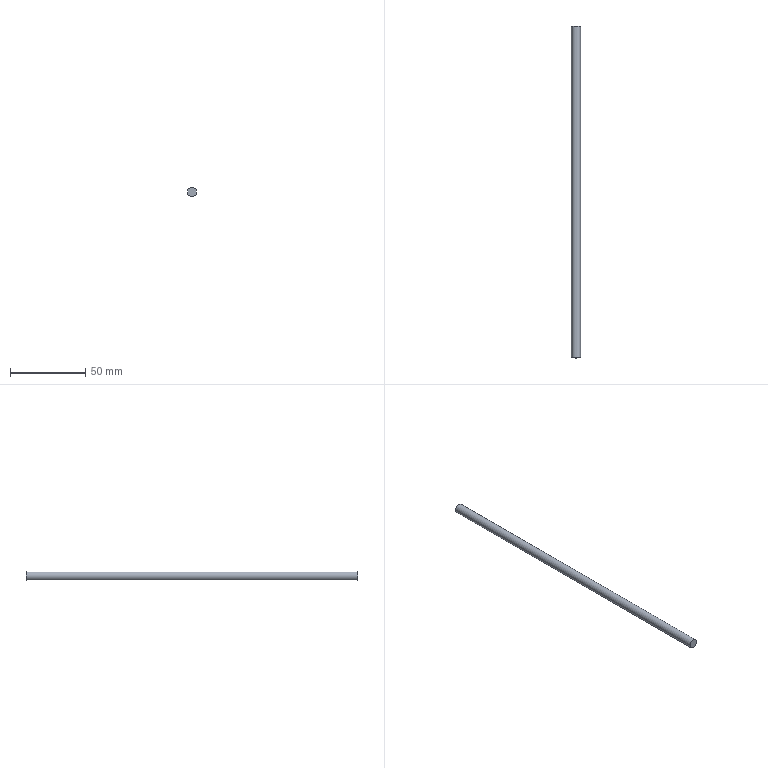Component | NX | HINGE | 1 solid | 3 faces | box 6 x 220 x 6 mm | volume 6220 mm3 | plane 2 | cylinder 1 | commonest cylinder face diameters 6 x1
STEP:
#1=CARTESIAN_POINT('',(0.,0.,0.));
#2=DIRECTION('',(0.,0.,1.));
#3=DIRECTION('',(1.,0.,0.));
#4=AXIS2_PLACEMENT_3D('',#1,#2,#3);
#5=CARTESIAN_POINT('',(115.,-110.,164.));
#6=VERTEX_POINT('',#5);
#7=CARTESIAN_POINT('',(112.,-110.,164.));
#8=DIRECTION('',(0.,-1.,0.));
#9=DIRECTION('',(1.,0.,0.));
#10=AXIS2_PLACEMENT_3D('',#7,#8,#9);
#11=CIRCLE('',#10,3.);
#12=CARTESIAN_POINT('',(112.,-110.,164.));
#13=DIRECTION('',(0.,1.,0.));
#14=DIRECTION('',(0.,0.,1.));
#15=AXIS2_PLACEMENT_3D('',#12,#13,#14);
#16=CYLINDRICAL_SURFACE('',#15,3.);
#17=CARTESIAN_POINT('',(7.854,0.));
#18=DIRECTION('',(-1.,0.));
#19=VECTOR('',#18,1.);
#20=LINE('',#17,#19);
#21=(GEOMETRIC_REPRESENTATION_CONTEXT(2)PARAMETRIC_REPRESENTATION_CONTEXT()REPRESENTATION_CONTEXT('',''));
#22=DEFINITIONAL_REPRESENTATION('',(#20),#21);
#23=PCURVE('',#16,#22);
#24=CARTESIAN_POINT('',(112.,-110.,164.));
#25=DIRECTION('',(0.,-1.,0.));
#26=DIRECTION('',(0.,0.,-1.));
#27=AXIS2_PLACEMENT_3D('',#24,#25,#26);
#28=PLANE('',#27);
#29=CARTESIAN_POINT('',(0.,0.));
#30=DIRECTION('',(0.,1.));
#31=AXIS2_PLACEMENT_2D('',#29,#30);
#32=CIRCLE('',#31,3.);
#33=(GEOMETRIC_REPRESENTATION_CONTEXT(2)PARAMETRIC_REPRESENTATION_CONTEXT()REPRESENTATION_CONTEXT('',''));
#34=DEFINITIONAL_REPRESENTATION('',(#32),#33);
#35=PCURVE('',#28,#34);
#36=SURFACE_CURVE('',#11,(#23,#35),.PCURVE_S1.);
#37=EDGE_CURVE('',#6,#6,#36,.T.);
#38=ORIENTED_EDGE('',*,*,#37,.F.);
#39=CARTESIAN_POINT('',(115.,110.,164.));
#40=VERTEX_POINT('',#39);
#41=CARTESIAN_POINT('',(115.,-110.,164.));
#42=CARTESIAN_POINT('',(115.,110.,164.));
#43=B_SPLINE_CURVE_WITH_KNOTS('',1,(#41,#42),.UNSPECIFIED.,.F.,.F.,(2,2),(0.,220.),.PIECEWISE_BEZIER_KNOTS.);
#44=CARTESIAN_POINT('',(7.854,0.));
#45=DIRECTION('',(0.,1.));
#46=VECTOR('',#45,1.);
#47=LINE('',#44,#46);
#48=(GEOMETRIC_REPRESENTATION_CONTEXT(2)PARAMETRIC_REPRESENTATION_CONTEXT()REPRESENTATION_CONTEXT('',''));
#49=DEFINITIONAL_REPRESENTATION('',(#47),#48);
#50=PCURVE('',#16,#49);
#51=CARTESIAN_POINT('',(1.571,0.));
#52=DIRECTION('',(0.,1.));
#53=VECTOR('',#52,1.);
#54=LINE('',#51,#53);
#55=(GEOMETRIC_REPRESENTATION_CONTEXT(2)PARAMETRIC_REPRESENTATION_CONTEXT()REPRESENTATION_CONTEXT('',''));
#56=DEFINITIONAL_REPRESENTATION('',(#54),#55);
#57=PCURVE('',#16,#56);
#58=SEAM_CURVE('',#43,(#50,#57),.PCURVE_S1.);
#59=EDGE_CURVE('',#6,#40,#58,.T.);
#60=ORIENTED_EDGE('',*,*,#59,.T.);
#61=CARTESIAN_POINT('',(112.,110.,164.));
#62=DIRECTION('',(0.,-1.,0.));
#63=DIRECTION('',(1.,0.,0.));
#64=AXIS2_PLACEMENT_3D('',#61,#62,#63);
#65=CIRCLE('',#64,3.);
#66=CARTESIAN_POINT('',(7.854,220.));
#67=DIRECTION('',(-1.,0.));
#68=VECTOR('',#67,1.);
#69=LINE('',#66,#68);
#70=(GEOMETRIC_REPRESENTATION_CONTEXT(2)PARAMETRIC_REPRESENTATION_CONTEXT()REPRESENTATION_CONTEXT('',''));
#71=DEFINITIONAL_REPRESENTATION('',(#69),#70);
#72=PCURVE('',#16,#71);
#73=CARTESIAN_POINT('',(112.,110.,164.));
#74=DIRECTION('',(0.,-1.,0.));
#75=DIRECTION('',(0.,0.,-1.));
#76=AXIS2_PLACEMENT_3D('',#73,#74,#75);
#77=PLANE('',#76);
#78=CARTESIAN_POINT('',(0.,0.));
#79=DIRECTION('',(0.,1.));
#80=AXIS2_PLACEMENT_2D('',#78,#79);
#81=CIRCLE('',#80,3.);
#82=(GEOMETRIC_REPRESENTATION_CONTEXT(2)PARAMETRIC_REPRESENTATION_CONTEXT()REPRESENTATION_CONTEXT('',''));
#83=DEFINITIONAL_REPRESENTATION('',(#81),#82);
#84=PCURVE('',#77,#83);
#85=SURFACE_CURVE('',#65,(#72,#84),.PCURVE_S1.);
#86=EDGE_CURVE('',#40,#40,#85,.T.);
#87=ORIENTED_EDGE('',*,*,#86,.T.);
#88=ORIENTED_EDGE('',*,*,#59,.F.);
#89=EDGE_LOOP('',(#38,#60,#87,#88));
#90=FACE_BOUND('',#89,.T.);
#91=ADVANCED_FACE('',(#90),#16,.T.);
#92=ORIENTED_EDGE('',*,*,#37,.T.);
#93=EDGE_LOOP('',(#92));
#94=FACE_BOUND('',#93,.T.);
#95=ADVANCED_FACE('',(#94),#28,.T.);
#96=ORIENTED_EDGE('',*,*,#86,.F.);
#97=EDGE_LOOP('',(#96));
#98=FACE_BOUND('',#97,.T.);
#99=ADVANCED_FACE('',(#98),#77,.F.);
#100=CLOSED_SHELL('',(#91,#95,#99));
#101=MANIFOLD_SOLID_BREP('',#100);
#102=(LENGTH_UNIT()NAMED_UNIT(*)SI_UNIT(.MILLI.,.METRE.));
#103=UNCERTAINTY_MEASURE_WITH_UNIT(LENGTH_MEASURE(0.00001),#102,'','');
#104=(NAMED_UNIT(*)PLANE_ANGLE_UNIT()SI_UNIT($,.RADIAN.));
#105=(NAMED_UNIT(*)SI_UNIT($,.STERADIAN.)SOLID_ANGLE_UNIT());
#106=(GEOMETRIC_REPRESENTATION_CONTEXT(3)GLOBAL_UNCERTAINTY_ASSIGNED_CONTEXT((#103))GLOBAL_UNIT_ASSIGNED_CONTEXT((#102,#104,#105))REPRESENTATION_CONTEXT('',''));
#107=ADVANCED_BREP_SHAPE_REPRESENTATION('',(#4,#101),#106);